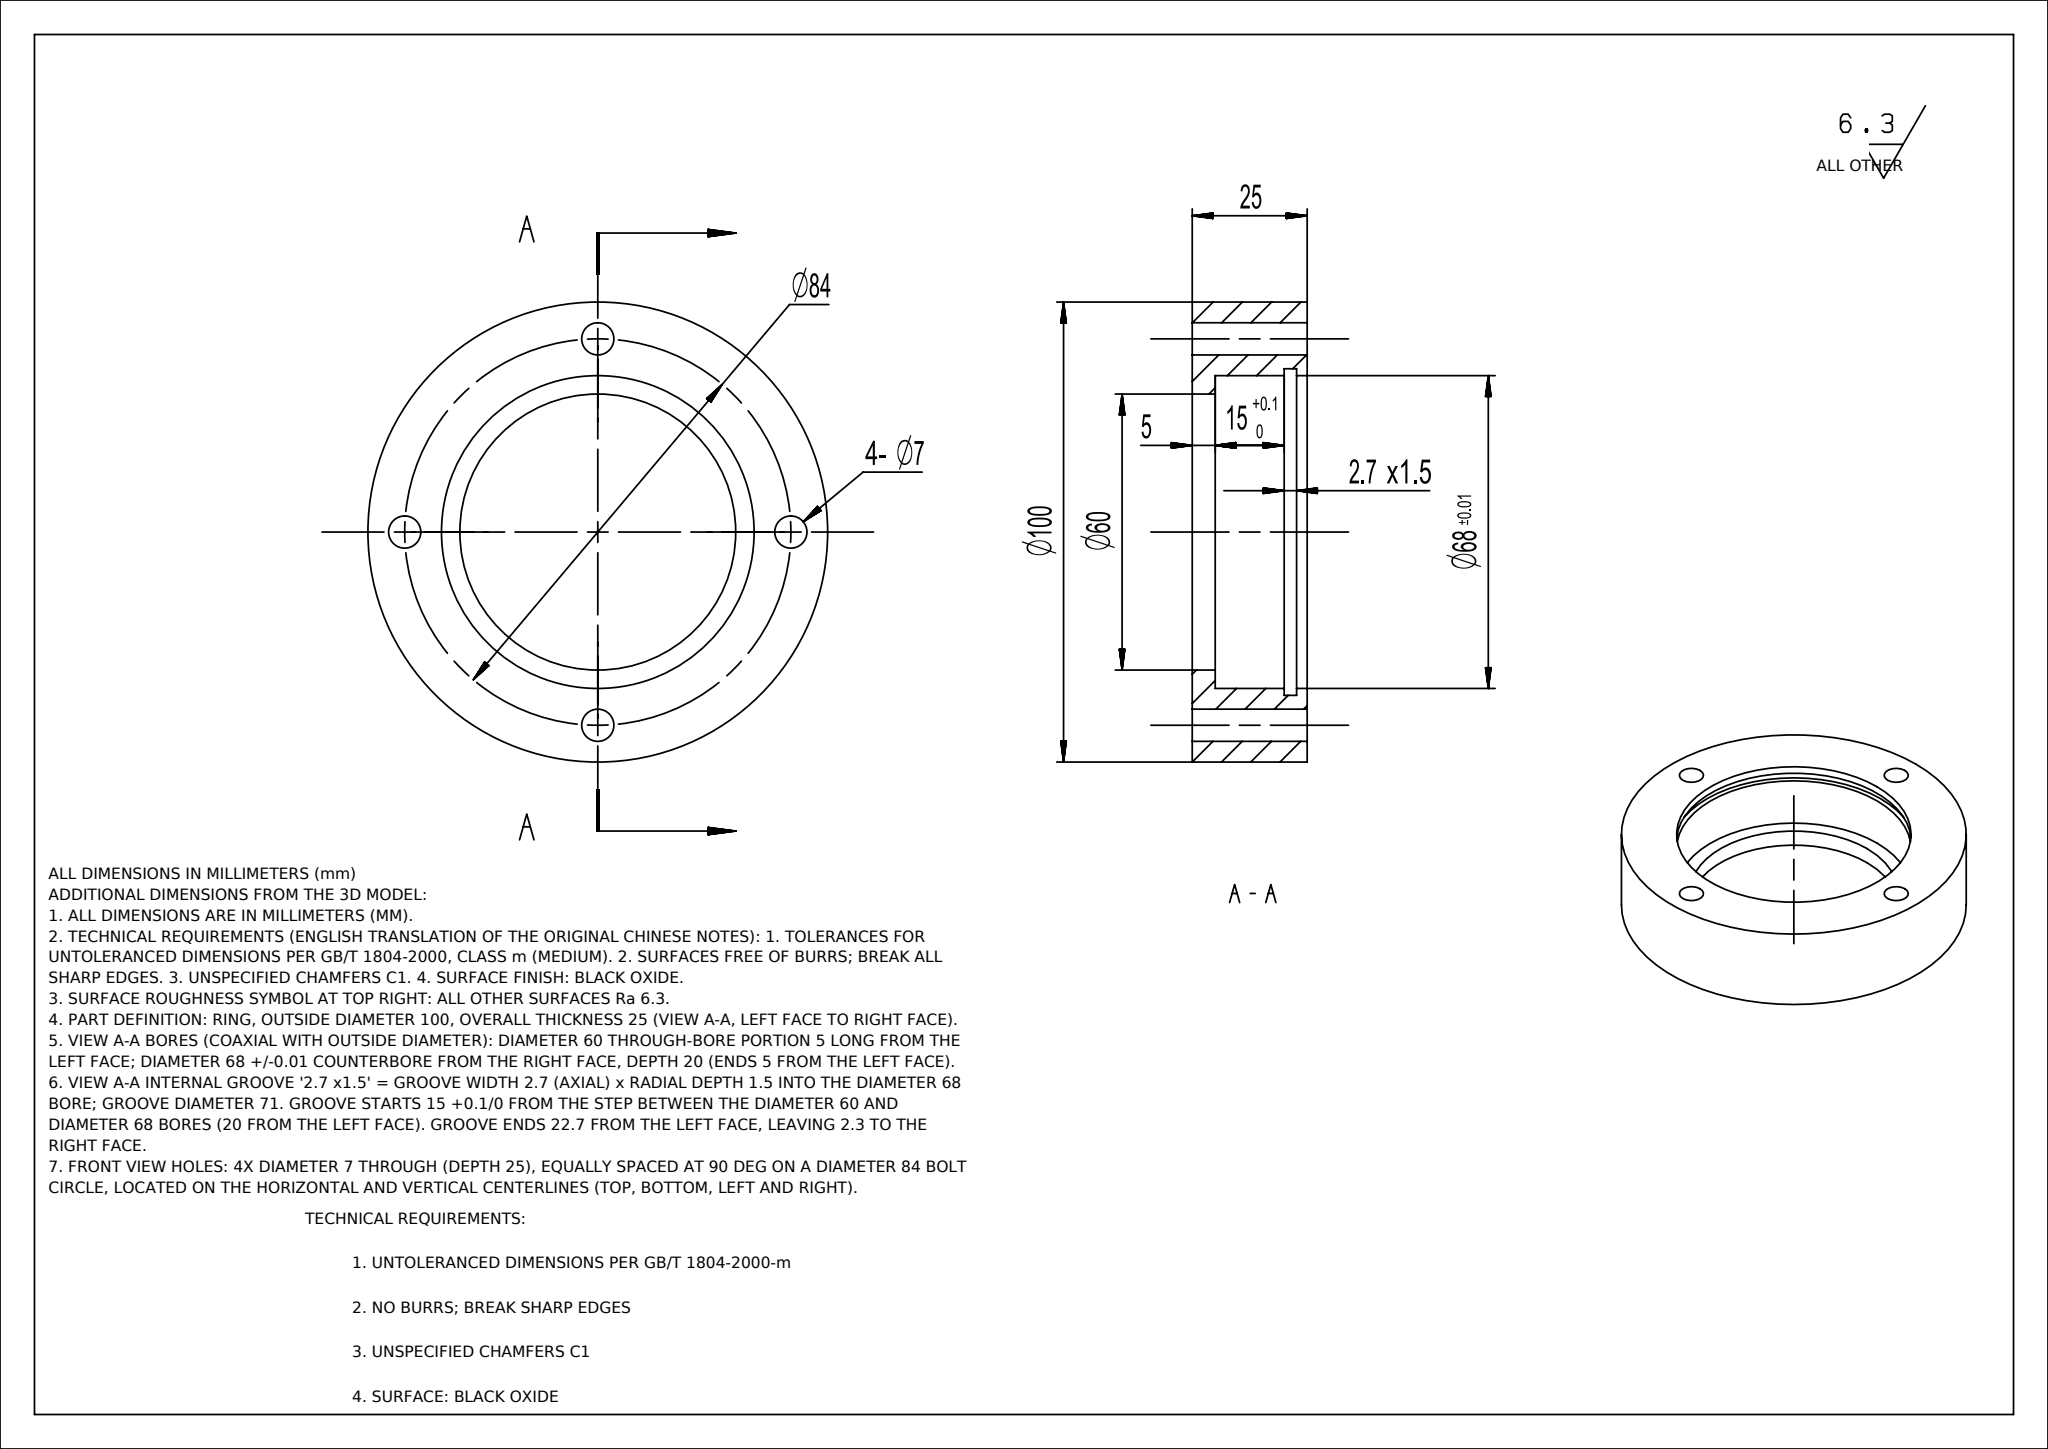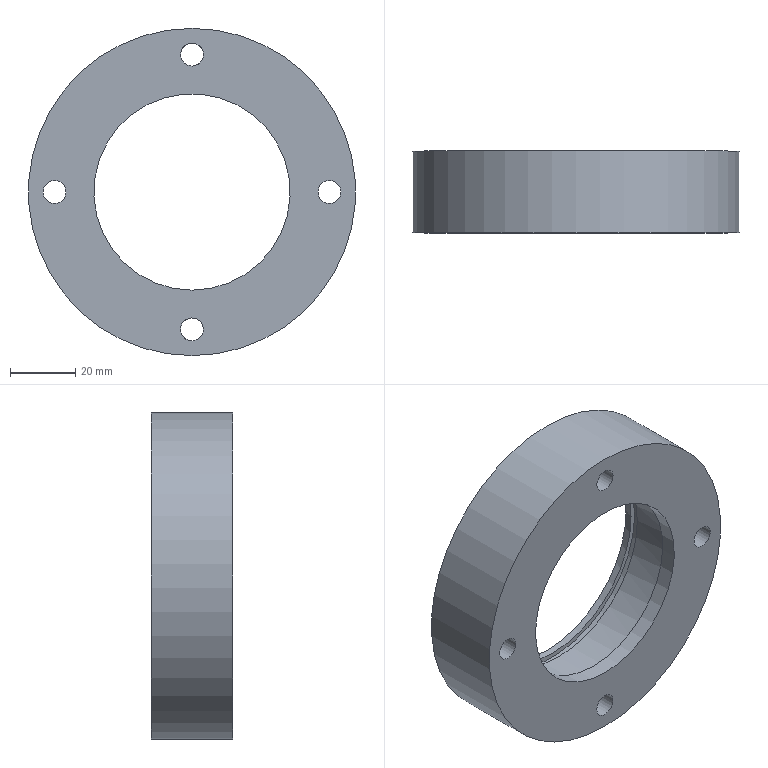Part | NX | mm | 1 solid | 14 faces | box 100 x 25 x 100 mm | volume 104846 mm3 | cylinder 9 | plane 5 | commonest cylinder face diameters 7 x4 68 x2 60 x1 100 x1 71 x1
STEP:
#1=CARTESIAN_POINT('',(0.,0.,0.));
#2=DIRECTION('',(0.,0.,1.));
#3=DIRECTION('',(1.,0.,0.));
#4=AXIS2_PLACEMENT_3D('',#1,#2,#3);
#5=(LENGTH_UNIT()NAMED_UNIT(*)SI_UNIT(.MILLI.,.METRE.));
#6=UNCERTAINTY_MEASURE_WITH_UNIT(LENGTH_MEASURE(0.00002),#5,'','');
#7=(NAMED_UNIT(*)PLANE_ANGLE_UNIT()SI_UNIT($,.RADIAN.));
#8=PLANE_ANGLE_MEASURE_WITH_UNIT(PLANE_ANGLE_MEASURE(0.01745),#7);
#9=DIMENSIONAL_EXPONENTS(0.,0.,0.,0.,0.,0.,0.);
#10=(CONVERSION_BASED_UNIT('',#8)NAMED_UNIT(#9)PLANE_ANGLE_UNIT());
#11=(NAMED_UNIT(*)SI_UNIT($,.STERADIAN.)SOLID_ANGLE_UNIT());
#12=(GEOMETRIC_REPRESENTATION_CONTEXT(3)GLOBAL_UNCERTAINTY_ASSIGNED_CONTEXT((#6))GLOBAL_UNIT_ASSIGNED_CONTEXT((#5,#10,#11))REPRESENTATION_CONTEXT('',''));
#13=SHAPE_REPRESENTATION('',(#4),#12);
#14=CARTESIAN_POINT('',(0.,5.,-34.));
#15=VERTEX_POINT('',#14);
#16=CARTESIAN_POINT('',(0.,5.,0.));
#17=DIRECTION('',(0.,-1.,0.));
#18=DIRECTION('',(0.,0.,-1.));
#19=AXIS2_PLACEMENT_3D('',#16,#17,#18);
#20=CIRCLE('',#19,34.);
#21=EDGE_CURVE('',#15,#15,#20,.T.);
#22=ORIENTED_EDGE('',*,*,#21,.T.);
#23=EDGE_LOOP('',(#22));
#24=FACE_BOUND('',#23,.T.);
#25=CARTESIAN_POINT('',(0.,20.,34.));
#26=VERTEX_POINT('',#25);
#27=CARTESIAN_POINT('',(0.,20.,0.));
#28=DIRECTION('',(0.,-1.,0.));
#29=DIRECTION('',(0.,0.,1.));
#30=AXIS2_PLACEMENT_3D('',#27,#28,#29);
#31=CIRCLE('',#30,34.);
#32=EDGE_CURVE('',#26,#26,#31,.T.);
#33=ORIENTED_EDGE('',*,*,#32,.F.);
#34=EDGE_LOOP('',(#33));
#35=FACE_BOUND('',#34,.T.);
#36=CARTESIAN_POINT('',(0.,0.,0.));
#37=DIRECTION('',(0.,-1.,0.));
#38=DIRECTION('',(0.,0.,-1.));
#39=AXIS2_PLACEMENT_3D('',#36,#37,#38);
#40=CYLINDRICAL_SURFACE('',#39,34.);
#41=ADVANCED_FACE('',(#24,#35),#40,.F.);
#42=CARTESIAN_POINT('',(3.5,-0.,42.));
#43=VERTEX_POINT('',#42);
#44=CARTESIAN_POINT('',(0.,-0.,42.));
#45=DIRECTION('',(0.,-1.,0.));
#46=DIRECTION('',(1.,0.,0.));
#47=AXIS2_PLACEMENT_3D('',#44,#45,#46);
#48=CIRCLE('',#47,3.5);
#49=EDGE_CURVE('',#43,#43,#48,.T.);
#50=ORIENTED_EDGE('',*,*,#49,.F.);
#51=EDGE_LOOP('',(#50));
#52=FACE_BOUND('',#51,.T.);
#53=CARTESIAN_POINT('',(-42.,-0.,3.5));
#54=VERTEX_POINT('',#53);
#55=CARTESIAN_POINT('',(-42.,-0.,0.));
#56=DIRECTION('',(0.,-1.,0.));
#57=DIRECTION('',(0.,0.,1.));
#58=AXIS2_PLACEMENT_3D('',#55,#56,#57);
#59=CIRCLE('',#58,3.5);
#60=EDGE_CURVE('',#54,#54,#59,.T.);
#61=ORIENTED_EDGE('',*,*,#60,.F.);
#62=EDGE_LOOP('',(#61));
#63=FACE_BOUND('',#62,.T.);
#64=CARTESIAN_POINT('',(-3.5,-0.,-42.));
#65=VERTEX_POINT('',#64);
#66=CARTESIAN_POINT('',(-0.,-0.,-42.));
#67=DIRECTION('',(0.,-1.,0.));
#68=DIRECTION('',(-1.,0.,0.));
#69=AXIS2_PLACEMENT_3D('',#66,#67,#68);
#70=CIRCLE('',#69,3.5);
#71=EDGE_CURVE('',#65,#65,#70,.T.);
#72=ORIENTED_EDGE('',*,*,#71,.F.);
#73=EDGE_LOOP('',(#72));
#74=FACE_BOUND('',#73,.T.);
#75=CARTESIAN_POINT('',(42.,-0.,-3.5));
#76=VERTEX_POINT('',#75);
#77=CARTESIAN_POINT('',(42.,-0.,-0.));
#78=DIRECTION('',(0.,-1.,0.));
#79=DIRECTION('',(0.,0.,-1.));
#80=AXIS2_PLACEMENT_3D('',#77,#78,#79);
#81=CIRCLE('',#80,3.5);
#82=EDGE_CURVE('',#76,#76,#81,.T.);
#83=ORIENTED_EDGE('',*,*,#82,.F.);
#84=EDGE_LOOP('',(#83));
#85=FACE_BOUND('',#84,.T.);
#86=CARTESIAN_POINT('',(0.,-0.,-30.));
#87=VERTEX_POINT('',#86);
#88=CARTESIAN_POINT('',(0.,-0.,0.));
#89=DIRECTION('',(0.,-1.,0.));
#90=DIRECTION('',(0.,0.,-1.));
#91=AXIS2_PLACEMENT_3D('',#88,#89,#90);
#92=CIRCLE('',#91,30.);
#93=EDGE_CURVE('',#87,#87,#92,.T.);
#94=ORIENTED_EDGE('',*,*,#93,.F.);
#95=EDGE_LOOP('',(#94));
#96=FACE_BOUND('',#95,.T.);
#97=CARTESIAN_POINT('',(0.,0.,-50.));
#98=VERTEX_POINT('',#97);
#99=CARTESIAN_POINT('',(0.,0.,0.));
#100=DIRECTION('',(0.,-1.,0.));
#101=DIRECTION('',(0.,0.,-1.));
#102=AXIS2_PLACEMENT_3D('',#99,#100,#101);
#103=CIRCLE('',#102,50.);
#104=EDGE_CURVE('',#98,#98,#103,.T.);
#105=ORIENTED_EDGE('',*,*,#104,.T.);
#106=EDGE_LOOP('',(#105));
#107=FACE_BOUND('',#106,.T.);
#108=CARTESIAN_POINT('',(0.,0.,50.));
#109=DIRECTION('',(0.,1.,0.));
#110=DIRECTION('',(0.,0.,1.));
#111=AXIS2_PLACEMENT_3D('',#108,#109,#110);
#112=PLANE('',#111);
#113=ADVANCED_FACE('',(#52,#63,#74,#85,#96,#107),#112,.F.);
#114=CARTESIAN_POINT('',(0.,5.,-30.));
#115=VERTEX_POINT('',#114);
#116=CARTESIAN_POINT('',(0.,5.,0.));
#117=DIRECTION('',(0.,-1.,0.));
#118=DIRECTION('',(0.,0.,-1.));
#119=AXIS2_PLACEMENT_3D('',#116,#117,#118);
#120=CIRCLE('',#119,30.);
#121=EDGE_CURVE('',#115,#115,#120,.T.);
#122=ORIENTED_EDGE('',*,*,#121,.F.);
#123=EDGE_LOOP('',(#122));
#124=FACE_BOUND('',#123,.T.);
#125=ORIENTED_EDGE('',*,*,#93,.T.);
#126=EDGE_LOOP('',(#125));
#127=FACE_BOUND('',#126,.T.);
#128=CARTESIAN_POINT('',(0.,0.,0.));
#129=DIRECTION('',(0.,-1.,0.));
#130=DIRECTION('',(0.,0.,-1.));
#131=AXIS2_PLACEMENT_3D('',#128,#129,#130);
#132=CYLINDRICAL_SURFACE('',#131,30.);
#133=ADVANCED_FACE('',(#124,#127),#132,.F.);
#134=ORIENTED_EDGE('',*,*,#21,.F.);
#135=EDGE_LOOP('',(#134));
#136=FACE_BOUND('',#135,.T.);
#137=ORIENTED_EDGE('',*,*,#121,.T.);
#138=EDGE_LOOP('',(#137));
#139=FACE_BOUND('',#138,.T.);
#140=CARTESIAN_POINT('',(0.,5.,30.));
#141=DIRECTION('',(0.,-1.,0.));
#142=DIRECTION('',(0.,0.,-1.));
#143=AXIS2_PLACEMENT_3D('',#140,#141,#142);
#144=PLANE('',#143);
#145=ADVANCED_FACE('',(#136,#139),#144,.F.);
#146=CARTESIAN_POINT('',(0.,22.7,34.));
#147=VERTEX_POINT('',#146);
#148=CARTESIAN_POINT('',(0.,22.7,0.));
#149=DIRECTION('',(0.,-1.,0.));
#150=DIRECTION('',(0.,0.,1.));
#151=AXIS2_PLACEMENT_3D('',#148,#149,#150);
#152=CIRCLE('',#151,34.);
#153=EDGE_CURVE('',#147,#147,#152,.T.);
#154=ORIENTED_EDGE('',*,*,#153,.T.);
#155=EDGE_LOOP('',(#154));
#156=FACE_BOUND('',#155,.T.);
#157=CARTESIAN_POINT('',(0.,25.,-34.));
#158=VERTEX_POINT('',#157);
#159=CARTESIAN_POINT('',(0.,25.,0.));
#160=DIRECTION('',(0.,-1.,0.));
#161=DIRECTION('',(0.,0.,-1.));
#162=AXIS2_PLACEMENT_3D('',#159,#160,#161);
#163=CIRCLE('',#162,34.);
#164=EDGE_CURVE('',#158,#158,#163,.T.);
#165=ORIENTED_EDGE('',*,*,#164,.F.);
#166=EDGE_LOOP('',(#165));
#167=FACE_BOUND('',#166,.T.);
#168=CARTESIAN_POINT('',(0.,0.,0.));
#169=DIRECTION('',(0.,-1.,0.));
#170=DIRECTION('',(0.,0.,-1.));
#171=AXIS2_PLACEMENT_3D('',#168,#169,#170);
#172=CYLINDRICAL_SURFACE('',#171,34.);
#173=ADVANCED_FACE('',(#156,#167),#172,.F.);
#174=CARTESIAN_POINT('',(0.,25.,38.5));
#175=VERTEX_POINT('',#174);
#176=CARTESIAN_POINT('',(0.,25.,42.));
#177=DIRECTION('',(0.,-1.,0.));
#178=DIRECTION('',(0.,0.,-1.));
#179=AXIS2_PLACEMENT_3D('',#176,#177,#178);
#180=CIRCLE('',#179,3.5);
#181=EDGE_CURVE('',#175,#175,#180,.T.);
#182=ORIENTED_EDGE('',*,*,#181,.T.);
#183=EDGE_LOOP('',(#182));
#184=FACE_BOUND('',#183,.T.);
#185=CARTESIAN_POINT('',(-42.,25.,-3.5));
#186=VERTEX_POINT('',#185);
#187=CARTESIAN_POINT('',(-42.,25.,0.));
#188=DIRECTION('',(0.,-1.,0.));
#189=DIRECTION('',(0.,0.,-1.));
#190=AXIS2_PLACEMENT_3D('',#187,#188,#189);
#191=CIRCLE('',#190,3.5);
#192=EDGE_CURVE('',#186,#186,#191,.T.);
#193=ORIENTED_EDGE('',*,*,#192,.T.);
#194=EDGE_LOOP('',(#193));
#195=FACE_BOUND('',#194,.T.);
#196=CARTESIAN_POINT('',(-0.,25.,-45.5));
#197=VERTEX_POINT('',#196);
#198=CARTESIAN_POINT('',(-0.,25.,-42.));
#199=DIRECTION('',(0.,-1.,0.));
#200=DIRECTION('',(0.,0.,-1.));
#201=AXIS2_PLACEMENT_3D('',#198,#199,#200);
#202=CIRCLE('',#201,3.5);
#203=EDGE_CURVE('',#197,#197,#202,.T.);
#204=ORIENTED_EDGE('',*,*,#203,.T.);
#205=EDGE_LOOP('',(#204));
#206=FACE_BOUND('',#205,.T.);
#207=CARTESIAN_POINT('',(42.,25.,-3.5));
#208=VERTEX_POINT('',#207);
#209=CARTESIAN_POINT('',(42.,25.,-0.));
#210=DIRECTION('',(0.,-1.,0.));
#211=DIRECTION('',(0.,0.,-1.));
#212=AXIS2_PLACEMENT_3D('',#209,#210,#211);
#213=CIRCLE('',#212,3.5);
#214=EDGE_CURVE('',#208,#208,#213,.T.);
#215=ORIENTED_EDGE('',*,*,#214,.T.);
#216=EDGE_LOOP('',(#215));
#217=FACE_BOUND('',#216,.T.);
#218=CARTESIAN_POINT('',(0.,25.,-50.));
#219=VERTEX_POINT('',#218);
#220=CARTESIAN_POINT('',(0.,25.,0.));
#221=DIRECTION('',(0.,-1.,0.));
#222=DIRECTION('',(0.,0.,-1.));
#223=AXIS2_PLACEMENT_3D('',#220,#221,#222);
#224=CIRCLE('',#223,50.);
#225=EDGE_CURVE('',#219,#219,#224,.T.);
#226=ORIENTED_EDGE('',*,*,#225,.F.);
#227=EDGE_LOOP('',(#226));
#228=FACE_BOUND('',#227,.T.);
#229=ORIENTED_EDGE('',*,*,#164,.T.);
#230=EDGE_LOOP('',(#229));
#231=FACE_BOUND('',#230,.T.);
#232=CARTESIAN_POINT('',(0.,25.,34.));
#233=DIRECTION('',(0.,-1.,0.));
#234=DIRECTION('',(0.,0.,-1.));
#235=AXIS2_PLACEMENT_3D('',#232,#233,#234);
#236=PLANE('',#235);
#237=ADVANCED_FACE('',(#184,#195,#206,#217,#228,#231),#236,.F.);
#238=ORIENTED_EDGE('',*,*,#104,.F.);
#239=EDGE_LOOP('',(#238));
#240=FACE_BOUND('',#239,.T.);
#241=ORIENTED_EDGE('',*,*,#225,.T.);
#242=EDGE_LOOP('',(#241));
#243=FACE_BOUND('',#242,.T.);
#244=CARTESIAN_POINT('',(0.,0.,0.));
#245=DIRECTION('',(0.,-1.,0.));
#246=DIRECTION('',(0.,0.,-1.));
#247=AXIS2_PLACEMENT_3D('',#244,#245,#246);
#248=CYLINDRICAL_SURFACE('',#247,50.);
#249=ADVANCED_FACE('',(#240,#243),#248,.T.);
#250=ORIENTED_EDGE('',*,*,#82,.T.);
#251=EDGE_LOOP('',(#250));
#252=FACE_BOUND('',#251,.T.);
#253=ORIENTED_EDGE('',*,*,#214,.F.);
#254=EDGE_LOOP('',(#253));
#255=FACE_BOUND('',#254,.T.);
#256=CARTESIAN_POINT('',(42.,320.,-0.));
#257=DIRECTION('',(0.,-1.,0.));
#258=DIRECTION('',(0.,0.,-1.));
#259=AXIS2_PLACEMENT_3D('',#256,#257,#258);
#260=CYLINDRICAL_SURFACE('',#259,3.5);
#261=ADVANCED_FACE('',(#252,#255),#260,.F.);
#262=ORIENTED_EDGE('',*,*,#71,.T.);
#263=EDGE_LOOP('',(#262));
#264=FACE_BOUND('',#263,.T.);
#265=ORIENTED_EDGE('',*,*,#203,.F.);
#266=EDGE_LOOP('',(#265));
#267=FACE_BOUND('',#266,.T.);
#268=CARTESIAN_POINT('',(-0.,320.,-42.));
#269=DIRECTION('',(0.,-1.,0.));
#270=DIRECTION('',(0.,0.,-1.));
#271=AXIS2_PLACEMENT_3D('',#268,#269,#270);
#272=CYLINDRICAL_SURFACE('',#271,3.5);
#273=ADVANCED_FACE('',(#264,#267),#272,.F.);
#274=ORIENTED_EDGE('',*,*,#60,.T.);
#275=EDGE_LOOP('',(#274));
#276=FACE_BOUND('',#275,.T.);
#277=ORIENTED_EDGE('',*,*,#192,.F.);
#278=EDGE_LOOP('',(#277));
#279=FACE_BOUND('',#278,.T.);
#280=CARTESIAN_POINT('',(-42.,320.,0.));
#281=DIRECTION('',(0.,-1.,0.));
#282=DIRECTION('',(0.,0.,-1.));
#283=AXIS2_PLACEMENT_3D('',#280,#281,#282);
#284=CYLINDRICAL_SURFACE('',#283,3.5);
#285=ADVANCED_FACE('',(#276,#279),#284,.F.);
#286=ORIENTED_EDGE('',*,*,#49,.T.);
#287=EDGE_LOOP('',(#286));
#288=FACE_BOUND('',#287,.T.);
#289=ORIENTED_EDGE('',*,*,#181,.F.);
#290=EDGE_LOOP('',(#289));
#291=FACE_BOUND('',#290,.T.);
#292=CARTESIAN_POINT('',(0.,320.,42.));
#293=DIRECTION('',(0.,-1.,0.));
#294=DIRECTION('',(0.,0.,-1.));
#295=AXIS2_PLACEMENT_3D('',#292,#293,#294);
#296=CYLINDRICAL_SURFACE('',#295,3.5);
#297=ADVANCED_FACE('',(#288,#291),#296,.F.);
#298=CARTESIAN_POINT('',(0.,20.,35.5));
#299=VERTEX_POINT('',#298);
#300=CARTESIAN_POINT('',(0.,20.,0.));
#301=DIRECTION('',(0.,-1.,0.));
#302=DIRECTION('',(0.,0.,1.));
#303=AXIS2_PLACEMENT_3D('',#300,#301,#302);
#304=CIRCLE('',#303,35.5);
#305=EDGE_CURVE('',#299,#299,#304,.T.);
#306=ORIENTED_EDGE('',*,*,#305,.F.);
#307=EDGE_LOOP('',(#306));
#308=FACE_BOUND('',#307,.T.);
#309=ORIENTED_EDGE('',*,*,#32,.T.);
#310=EDGE_LOOP('',(#309));
#311=FACE_BOUND('',#310,.T.);
#312=CARTESIAN_POINT('',(0.,20.,0.));
#313=DIRECTION('',(0.,1.,0.));
#314=DIRECTION('',(0.,0.,1.));
#315=AXIS2_PLACEMENT_3D('',#312,#313,#314);
#316=PLANE('',#315);
#317=ADVANCED_FACE('',(#308,#311),#316,.T.);
#318=CARTESIAN_POINT('',(0.,22.7,35.5));
#319=VERTEX_POINT('',#318);
#320=CARTESIAN_POINT('',(0.,22.7,0.));
#321=DIRECTION('',(0.,-1.,0.));
#322=DIRECTION('',(0.,0.,1.));
#323=AXIS2_PLACEMENT_3D('',#320,#321,#322);
#324=CIRCLE('',#323,35.5);
#325=EDGE_CURVE('',#319,#319,#324,.T.);
#326=ORIENTED_EDGE('',*,*,#325,.T.);
#327=EDGE_LOOP('',(#326));
#328=FACE_BOUND('',#327,.T.);
#329=ORIENTED_EDGE('',*,*,#153,.F.);
#330=EDGE_LOOP('',(#329));
#331=FACE_BOUND('',#330,.T.);
#332=CARTESIAN_POINT('',(0.,22.7,0.));
#333=DIRECTION('',(0.,1.,0.));
#334=DIRECTION('',(0.,0.,1.));
#335=AXIS2_PLACEMENT_3D('',#332,#333,#334);
#336=PLANE('',#335);
#337=ADVANCED_FACE('',(#328,#331),#336,.F.);
#338=ORIENTED_EDGE('',*,*,#325,.F.);
#339=EDGE_LOOP('',(#338));
#340=FACE_BOUND('',#339,.T.);
#341=ORIENTED_EDGE('',*,*,#305,.T.);
#342=EDGE_LOOP('',(#341));
#343=FACE_BOUND('',#342,.T.);
#344=CARTESIAN_POINT('',(0.,21.35,0.));
#345=DIRECTION('',(0.,1.,0.));
#346=DIRECTION('',(0.,0.,1.));
#347=AXIS2_PLACEMENT_3D('',#344,#345,#346);
#348=CYLINDRICAL_SURFACE('',#347,35.5);
#349=ADVANCED_FACE('',(#340,#343),#348,.F.);
#350=CLOSED_SHELL('',(#41,#113,#133,#145,#173,#237,#249,#261,#273,#285,#297,#317,#337,#349));
#351=MANIFOLD_SOLID_BREP('',#350);
#352=ADVANCED_BREP_SHAPE_REPRESENTATION('',(#351),#12);
#353=SHAPE_REPRESENTATION_RELATIONSHIP('','',#13,#352);
#354=PRESENTATION_LAYER_ASSIGNMENT('','',(#351));
#355=COLOUR_RGB('',0.4,0.4,0.4);
#356=FILL_AREA_STYLE_COLOUR('',#355);
#357=FILL_AREA_STYLE('',(#356));
#358=SURFACE_STYLE_FILL_AREA(#357);
#359=SURFACE_SIDE_STYLE('',(#358));
#360=SURFACE_STYLE_USAGE(.BOTH.,#359);
#361=PRESENTATION_STYLE_ASSIGNMENT((#360));
#362=STYLED_ITEM('',(#361),#351);
#363=MECHANICAL_DESIGN_GEOMETRIC_PRESENTATION_REPRESENTATION('',(#362),#12);